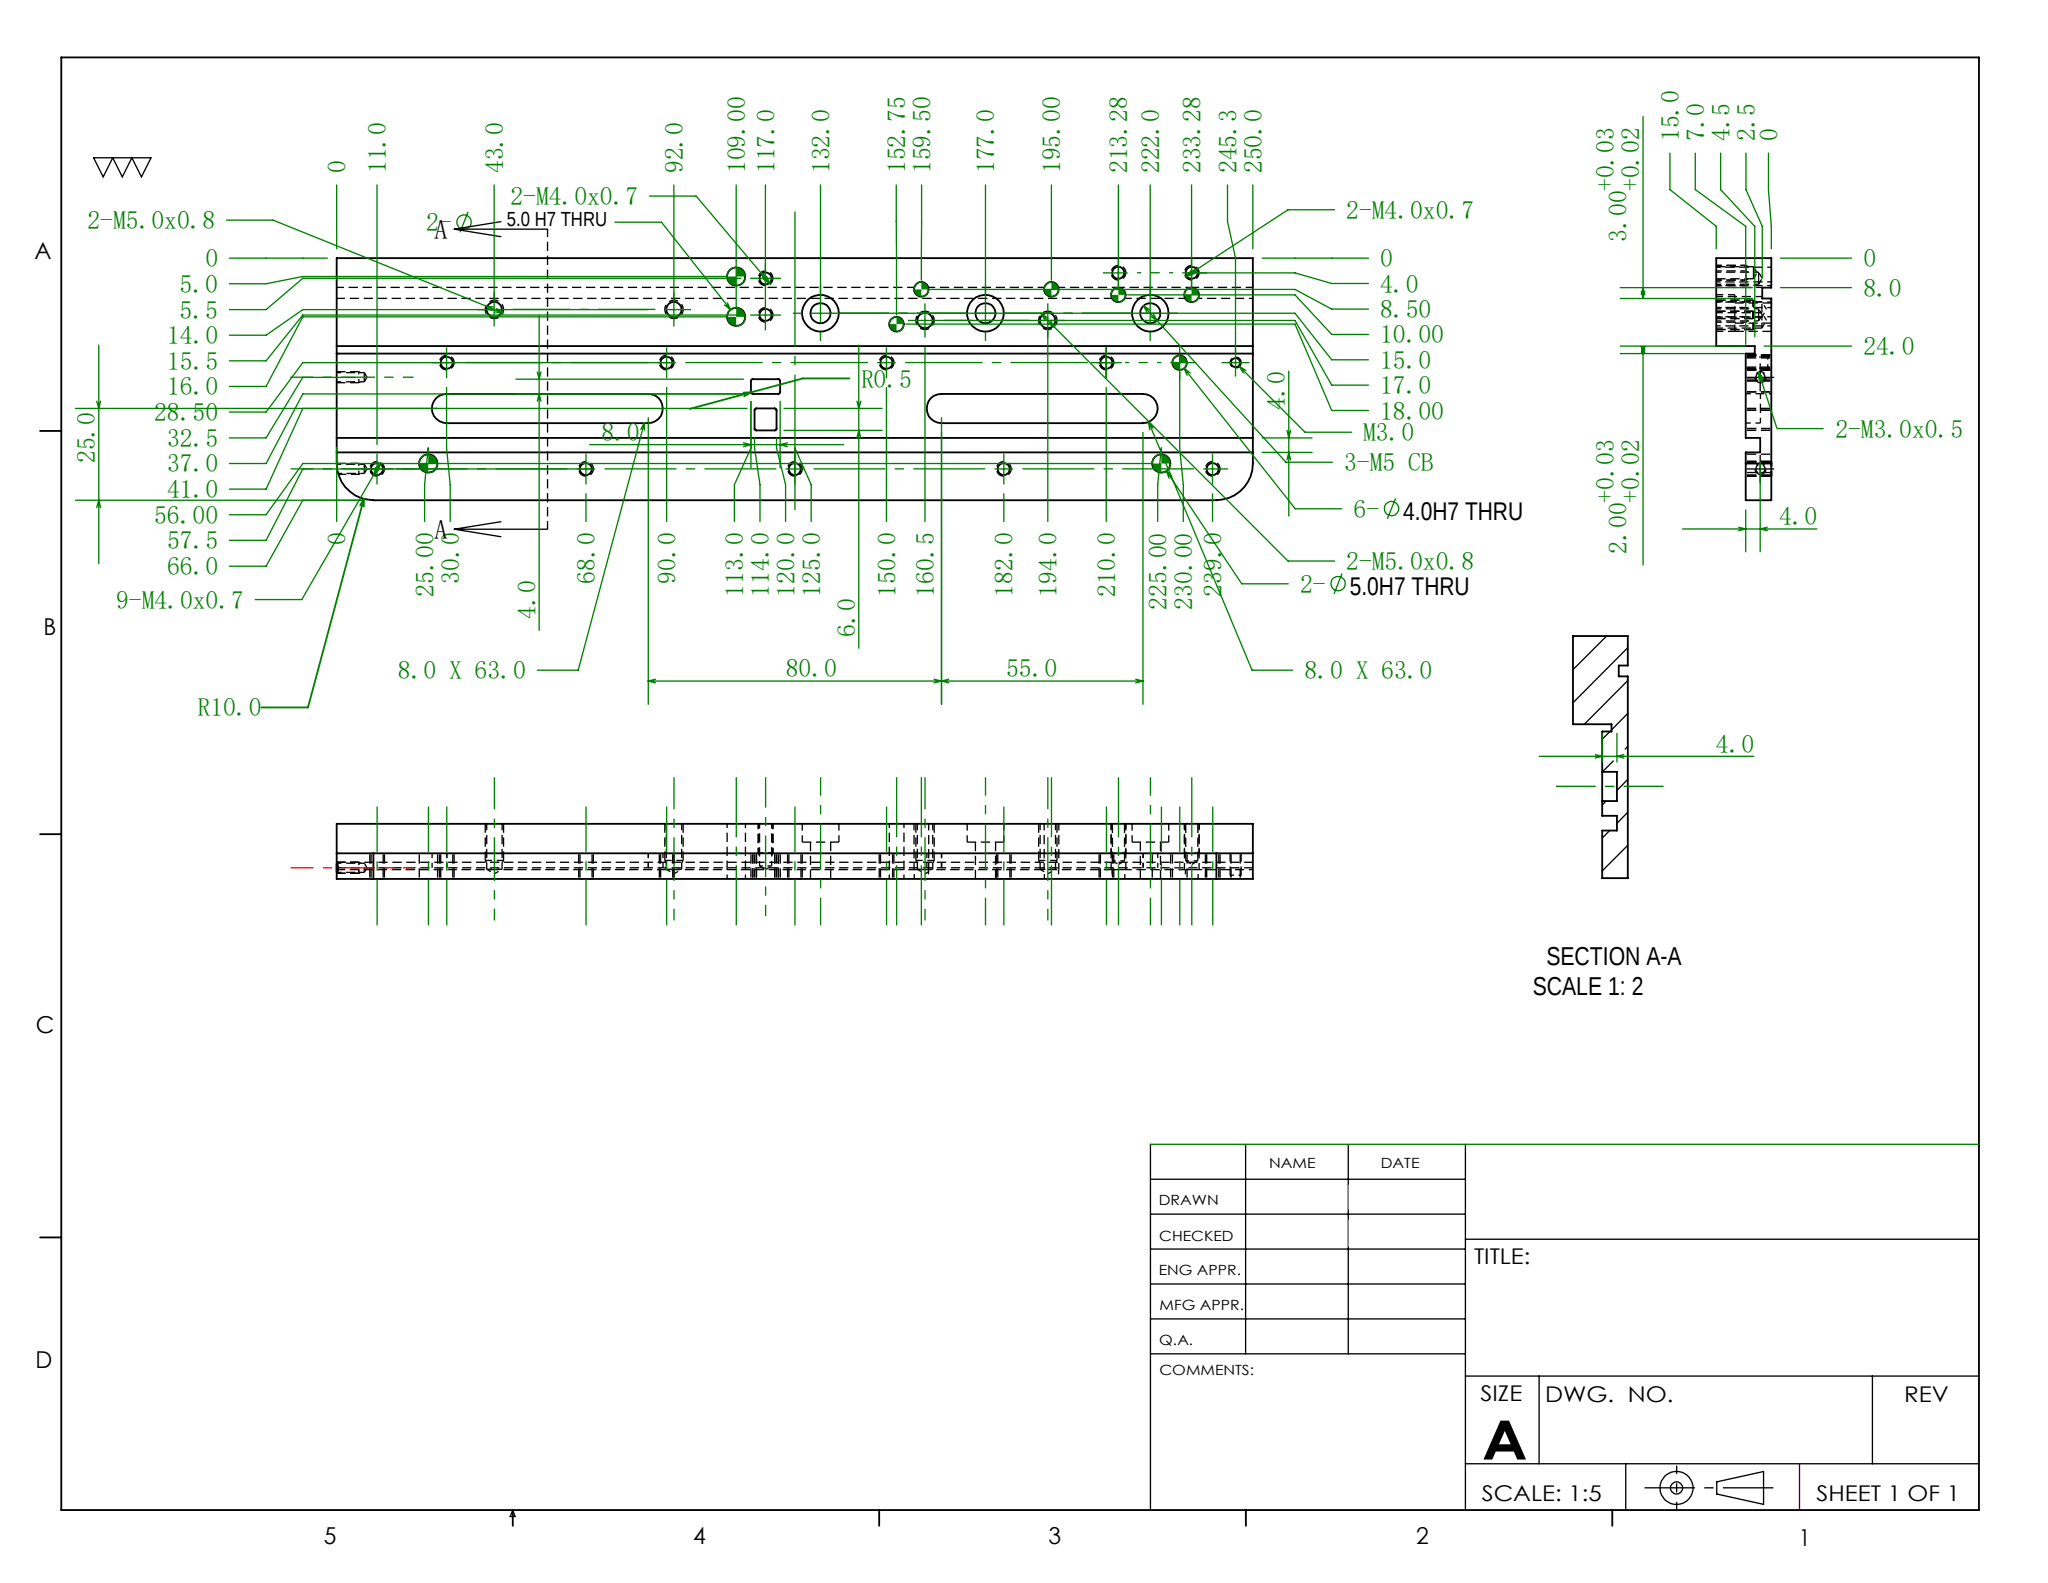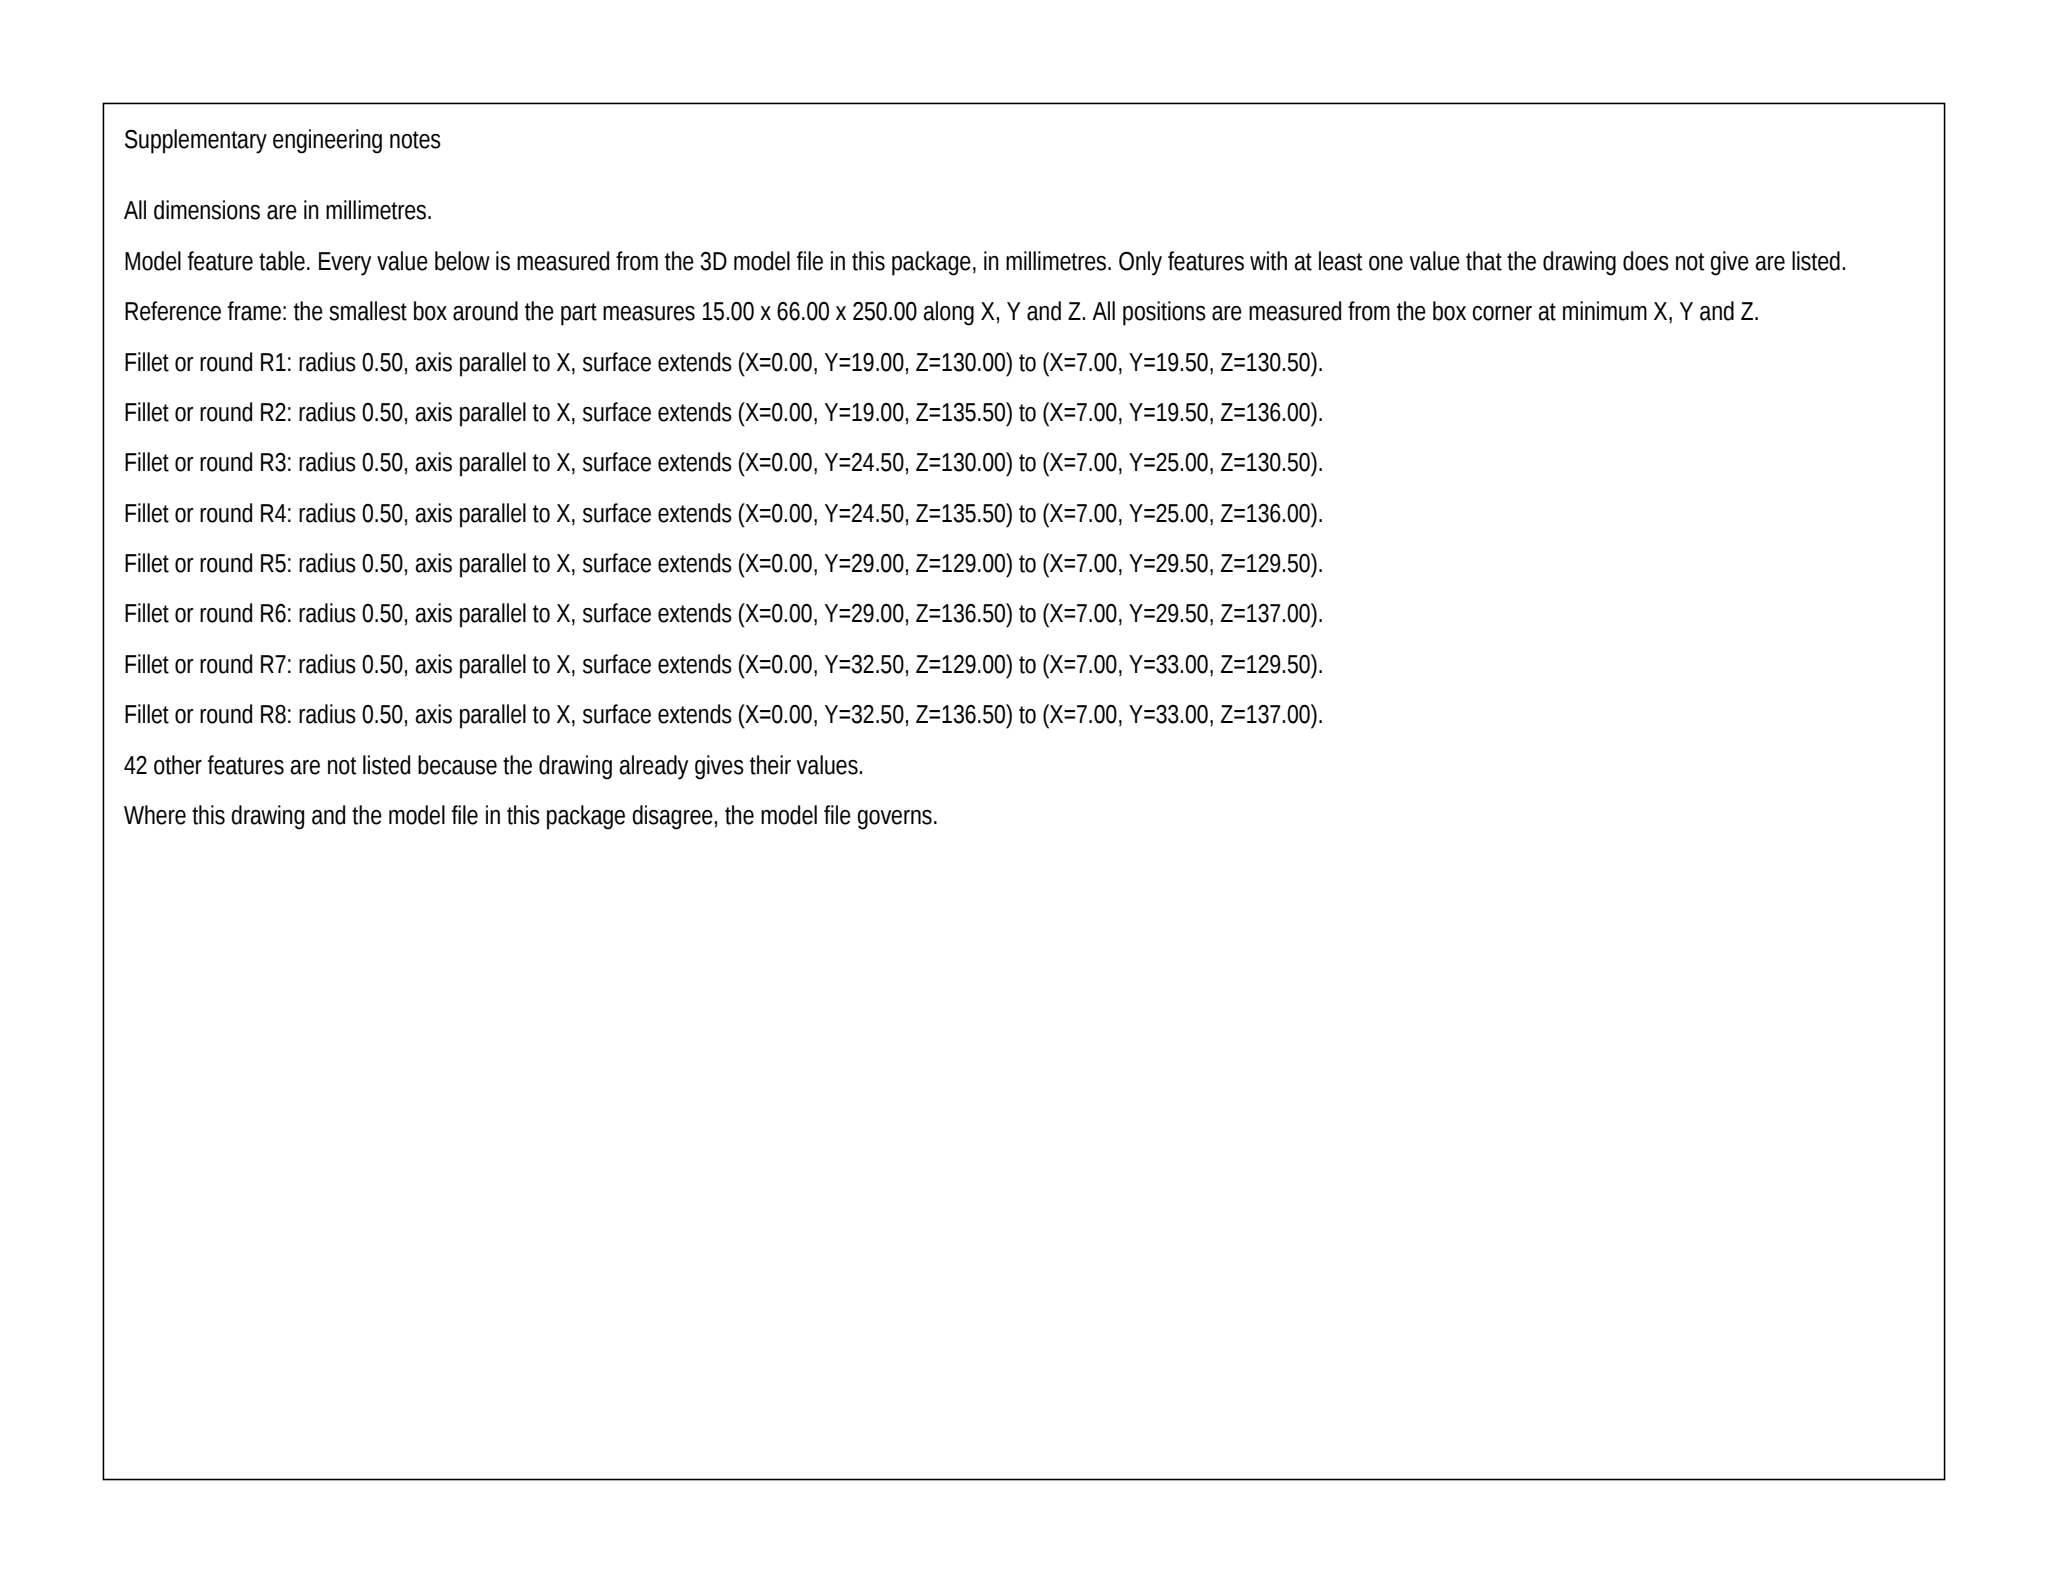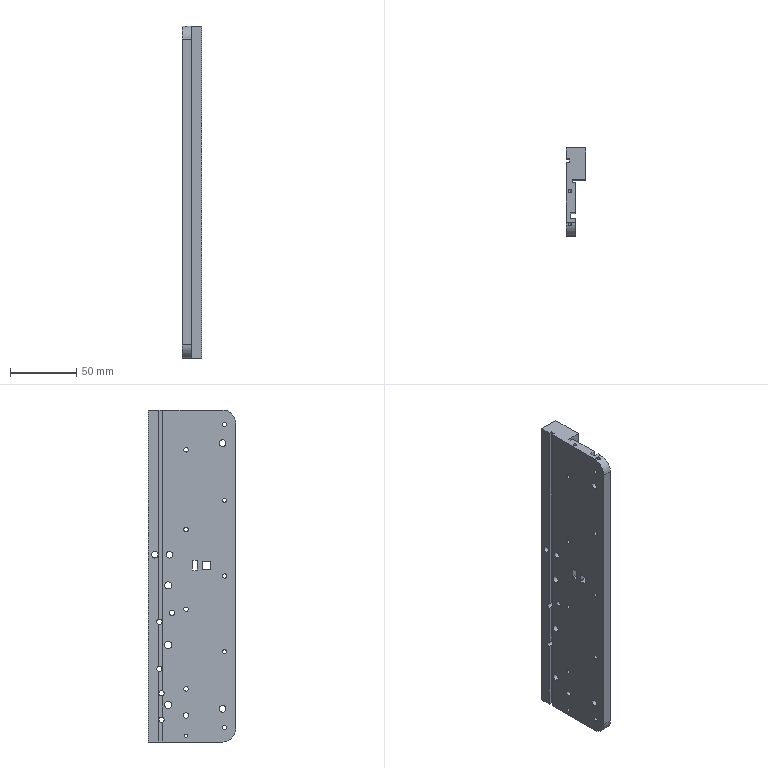Part | SolidWorks | mm | 1 solid | 149 faces | box 15 x 66 x 250 mm | volume 146246 mm3 | cylinder 88 | plane 41 | cone 20 | commonest cylinder face diameters 3.3 x26 4 x12 5 x8 4.2 x8 1 x8 8 x6 2.5 x6 10 x6